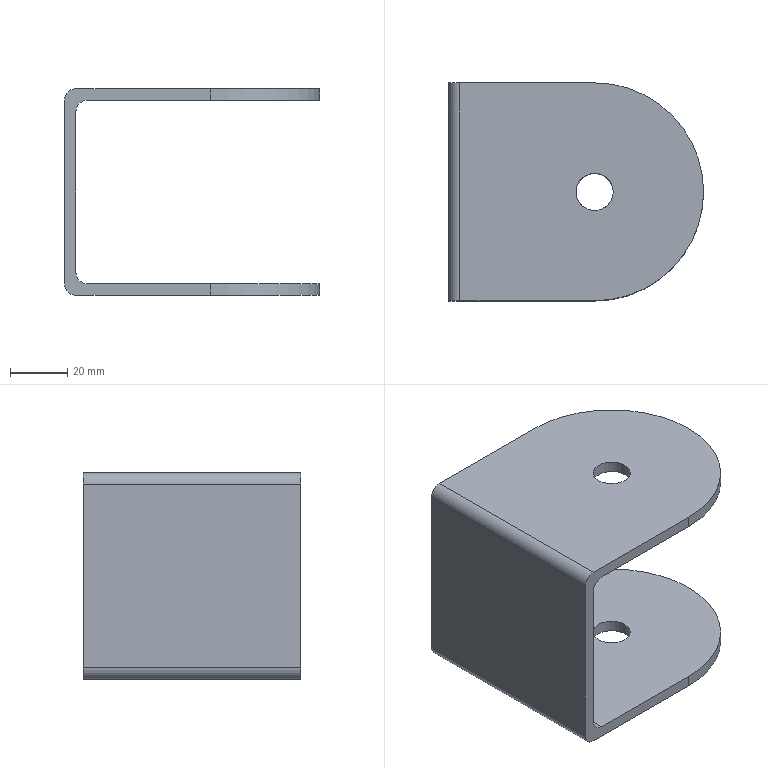Component | NX | BASE_FRAME_CONN | 1 solid | 18 faces | volume 67548 mm3 | cylinder 10 | plane 8 | commonest cylinder face diameters 76 x4 8 x4 13 x2